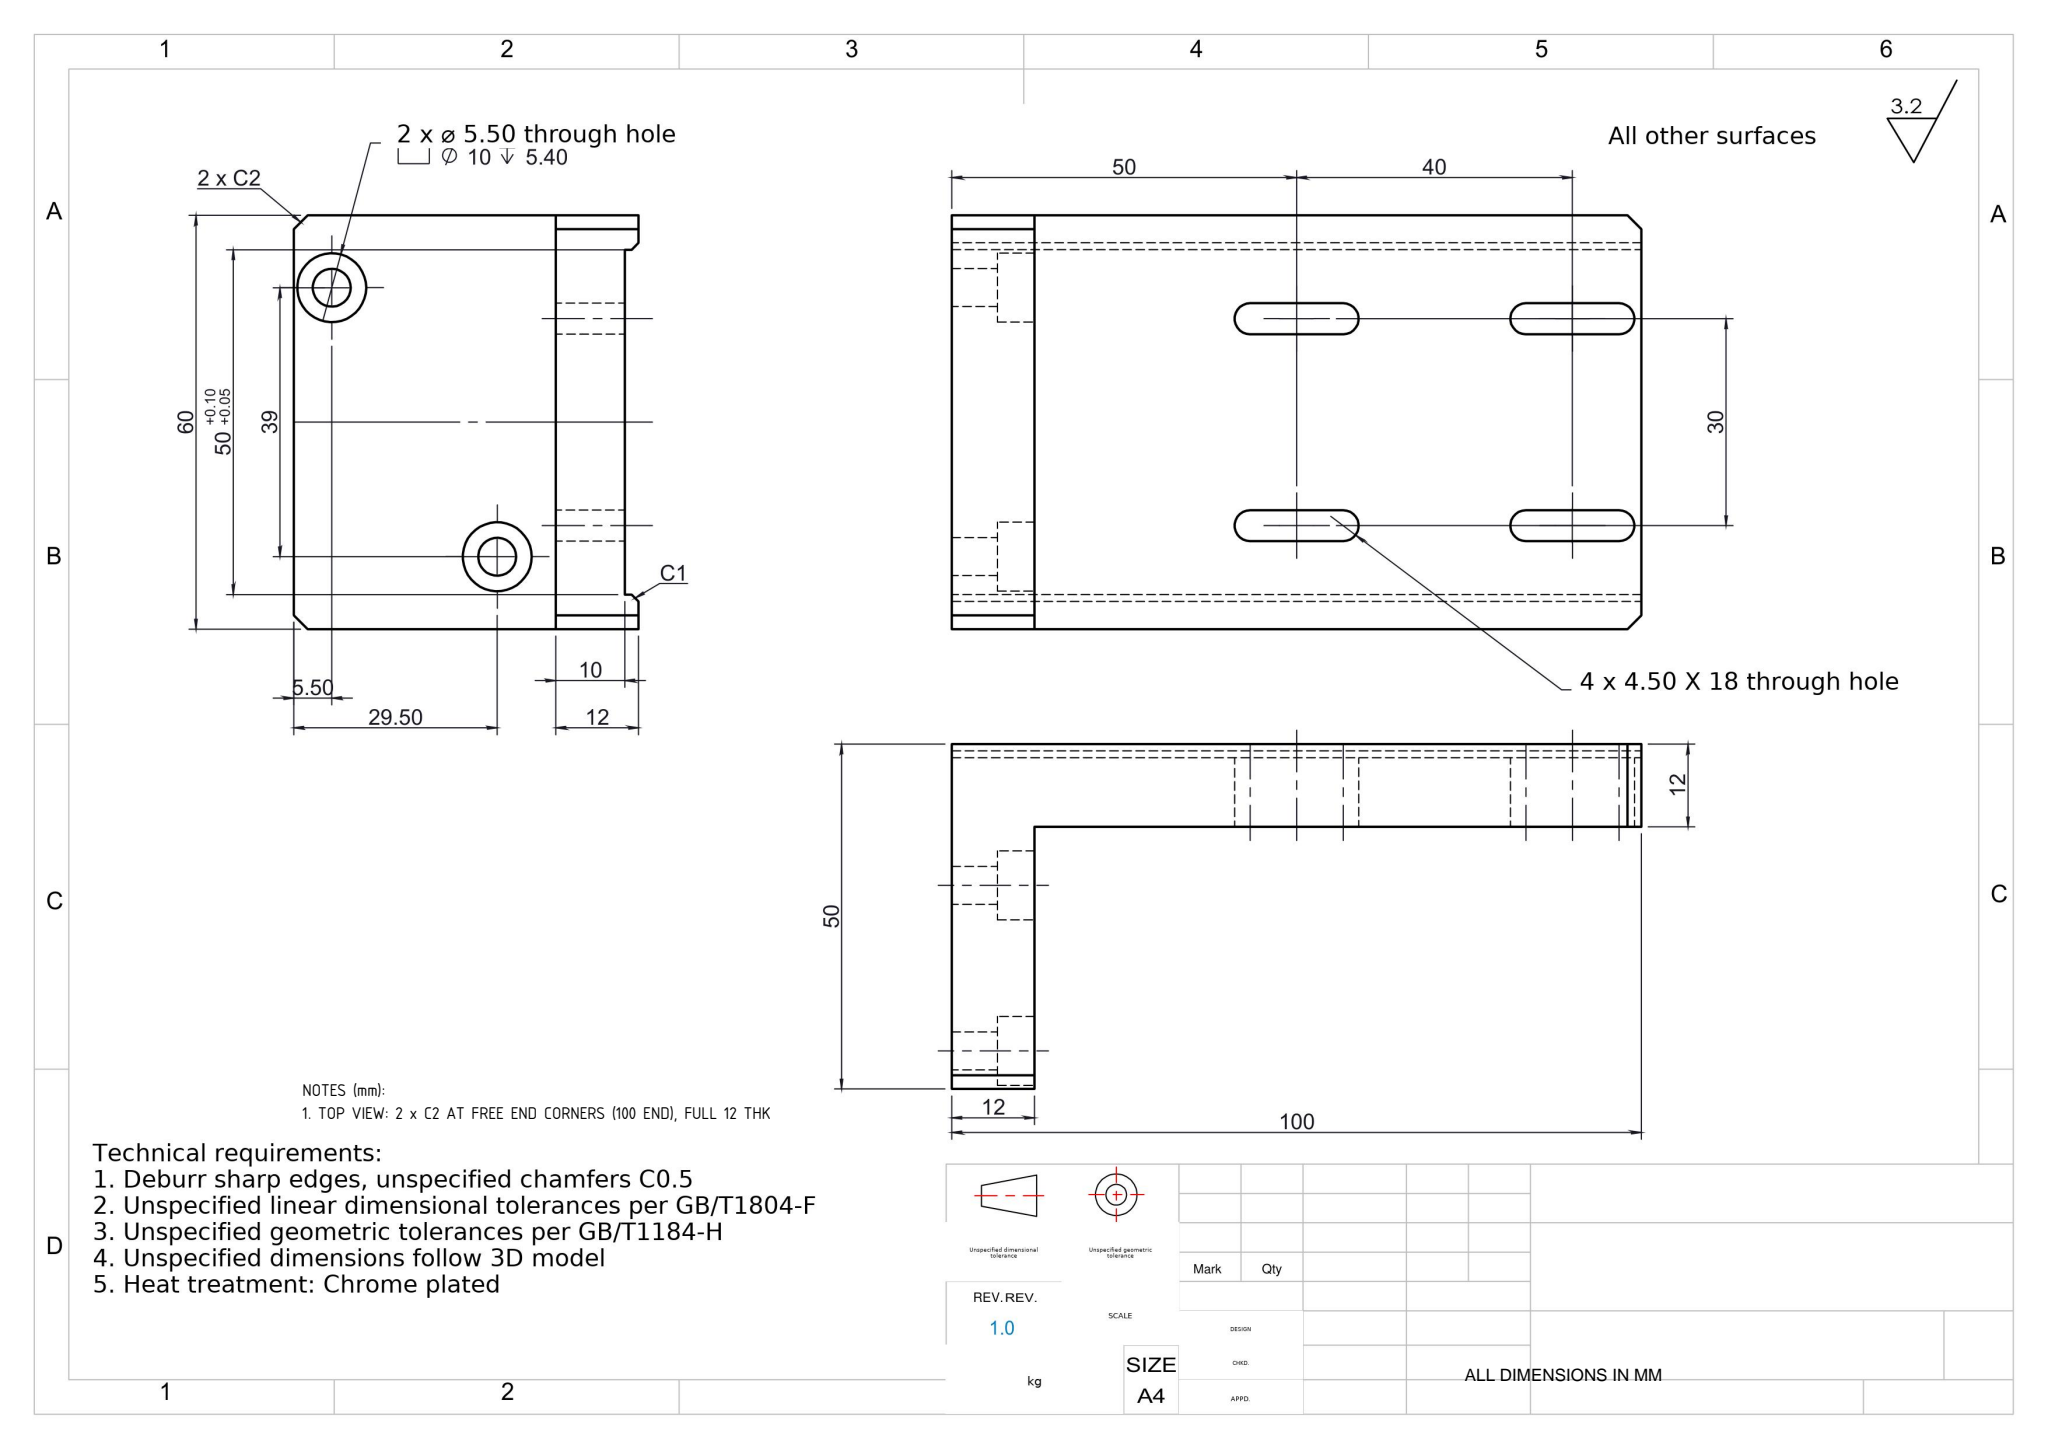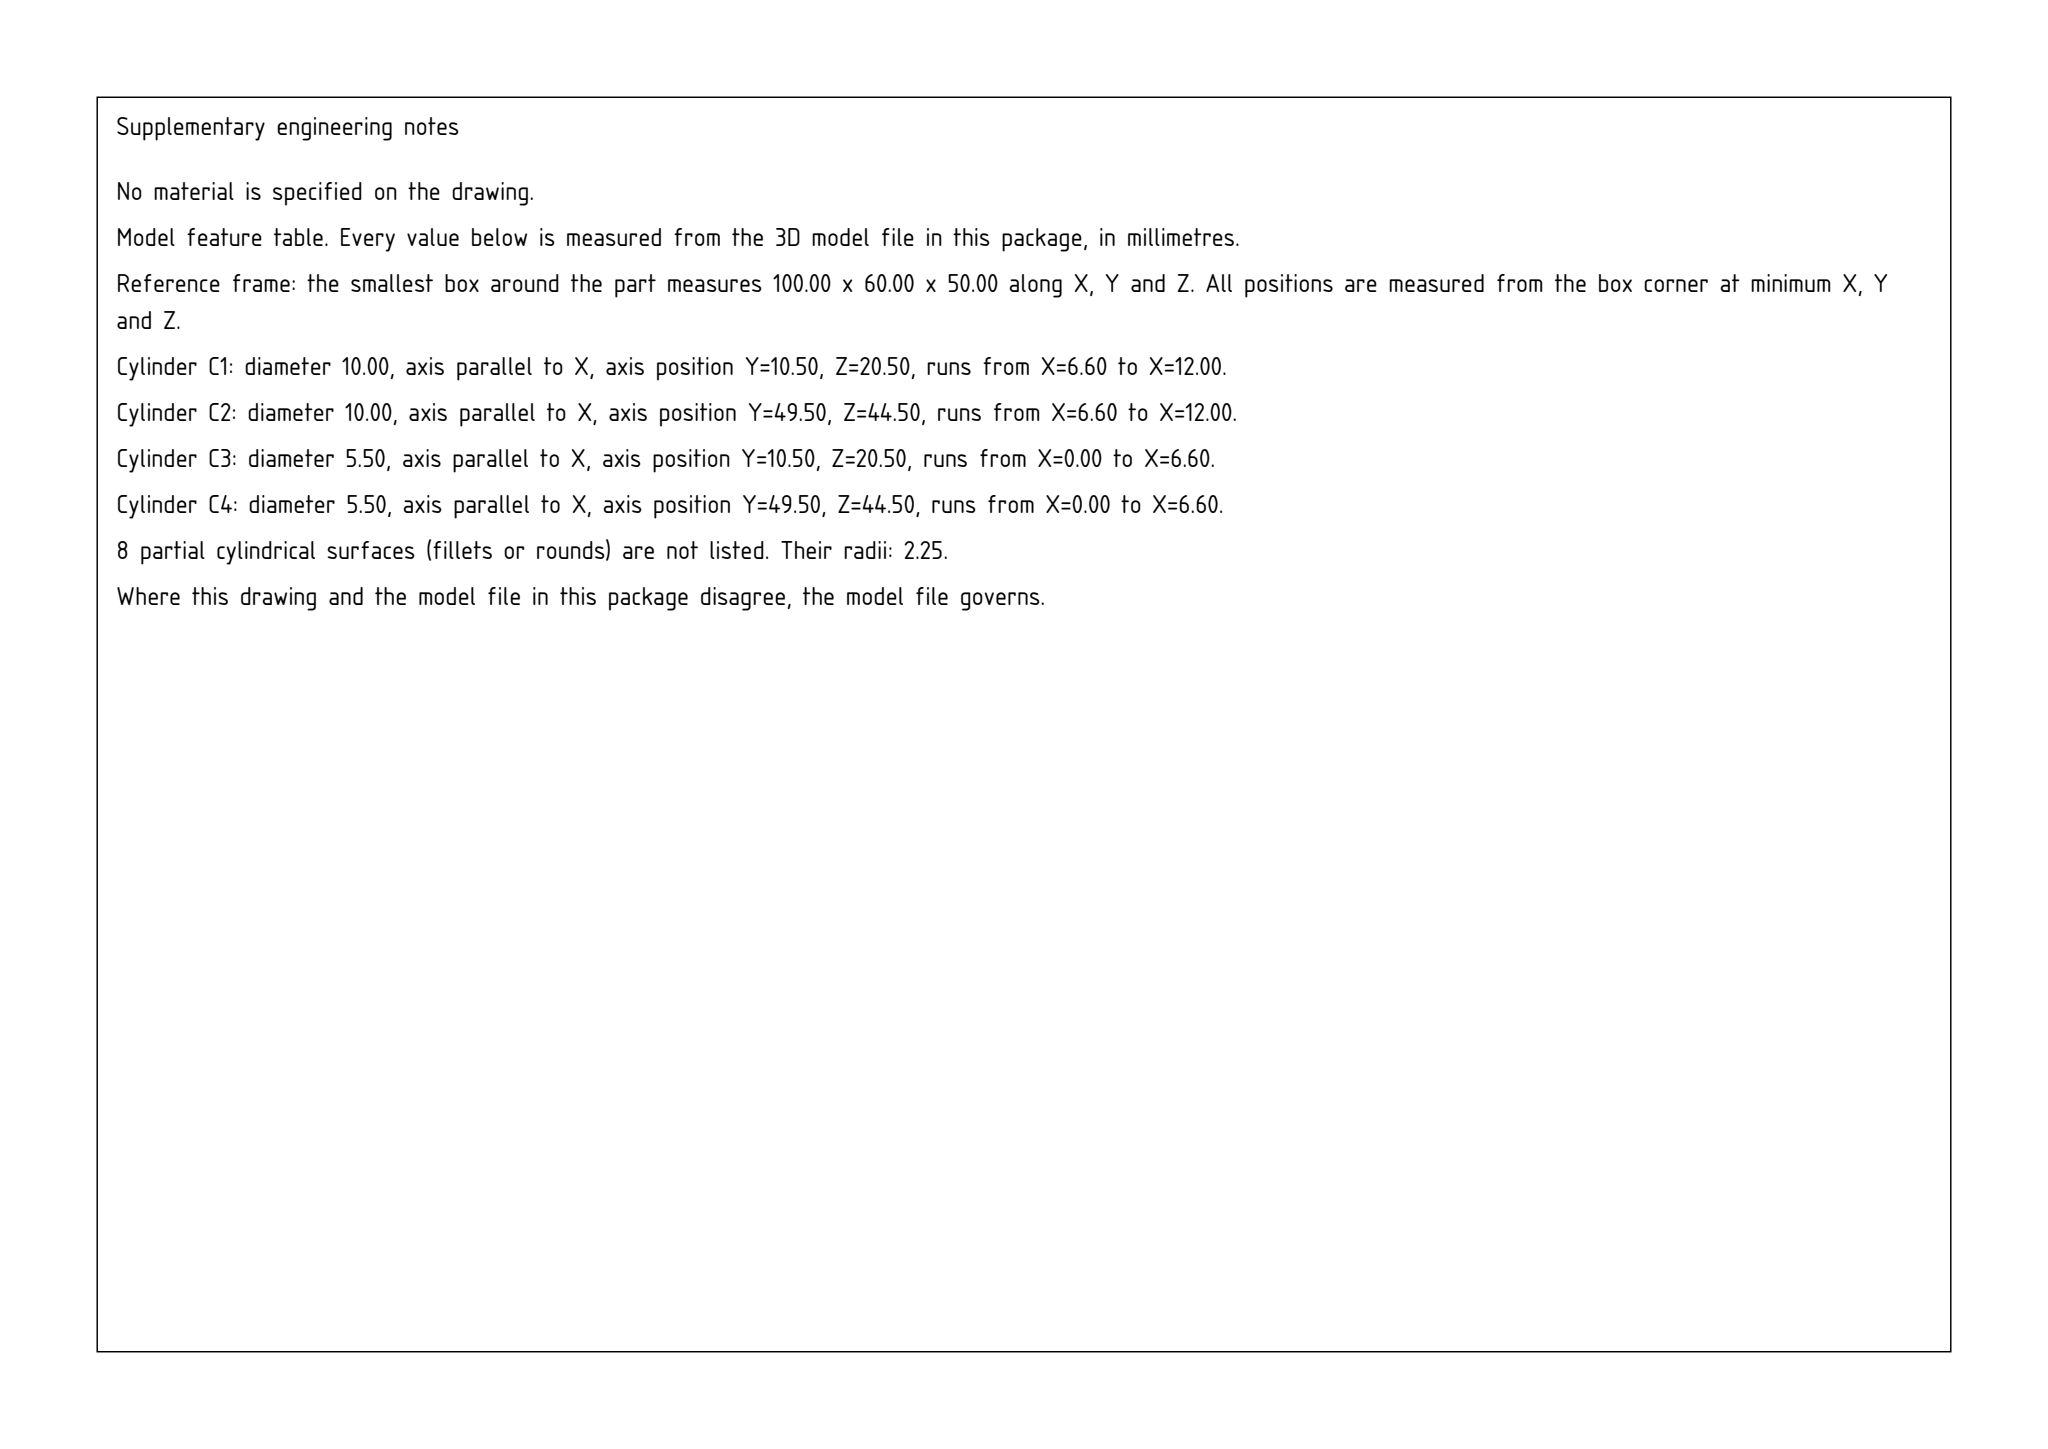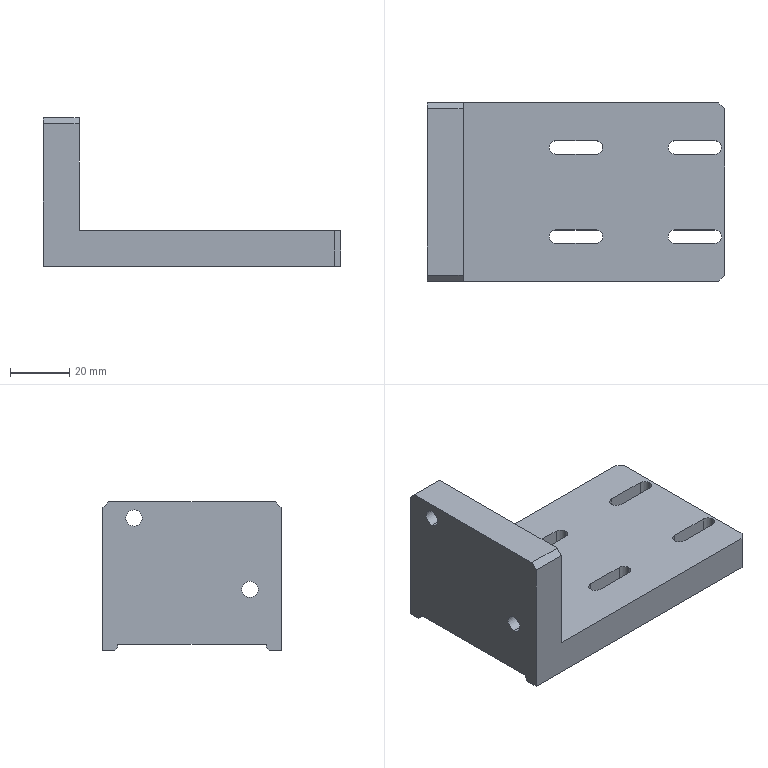Part | SolidWorks | mm | 1 solid | 48 faces | box 100 x 60 x 50 mm | volume 84936 mm3 | plane 28 | cylinder 20 | commonest cylinder face diameters 4.5 x12 10 x4 5.5 x4
Drawing notes:
TOP VIEW: 2 x C2 AT FREE END CORNERS (100 END), FULL 12 THK | from the solid: inclined_planes 45/45/90 at bbox_from [98,0,0] and [98,58,0], size [2,2,12] -> 2x2 chamfer thru 12 thk at x=100 end